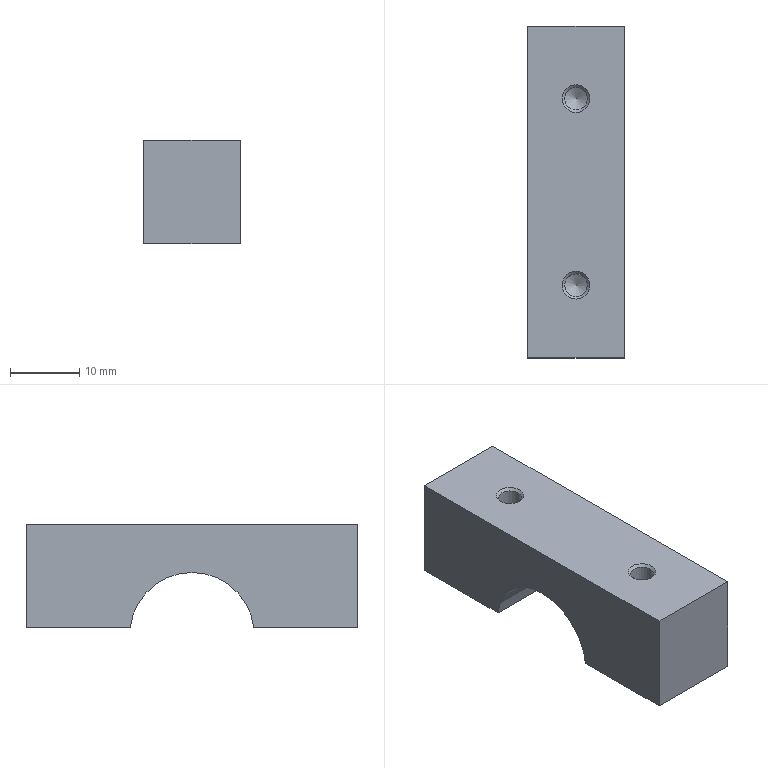Component | NX | UPPER_CONN_PLATE | 1 solid | 20 faces | volume 8194 mm3 | cone 8 | plane 7 | cylinder 5 | commonest cylinder face diameters 3.3 x4 18 x1